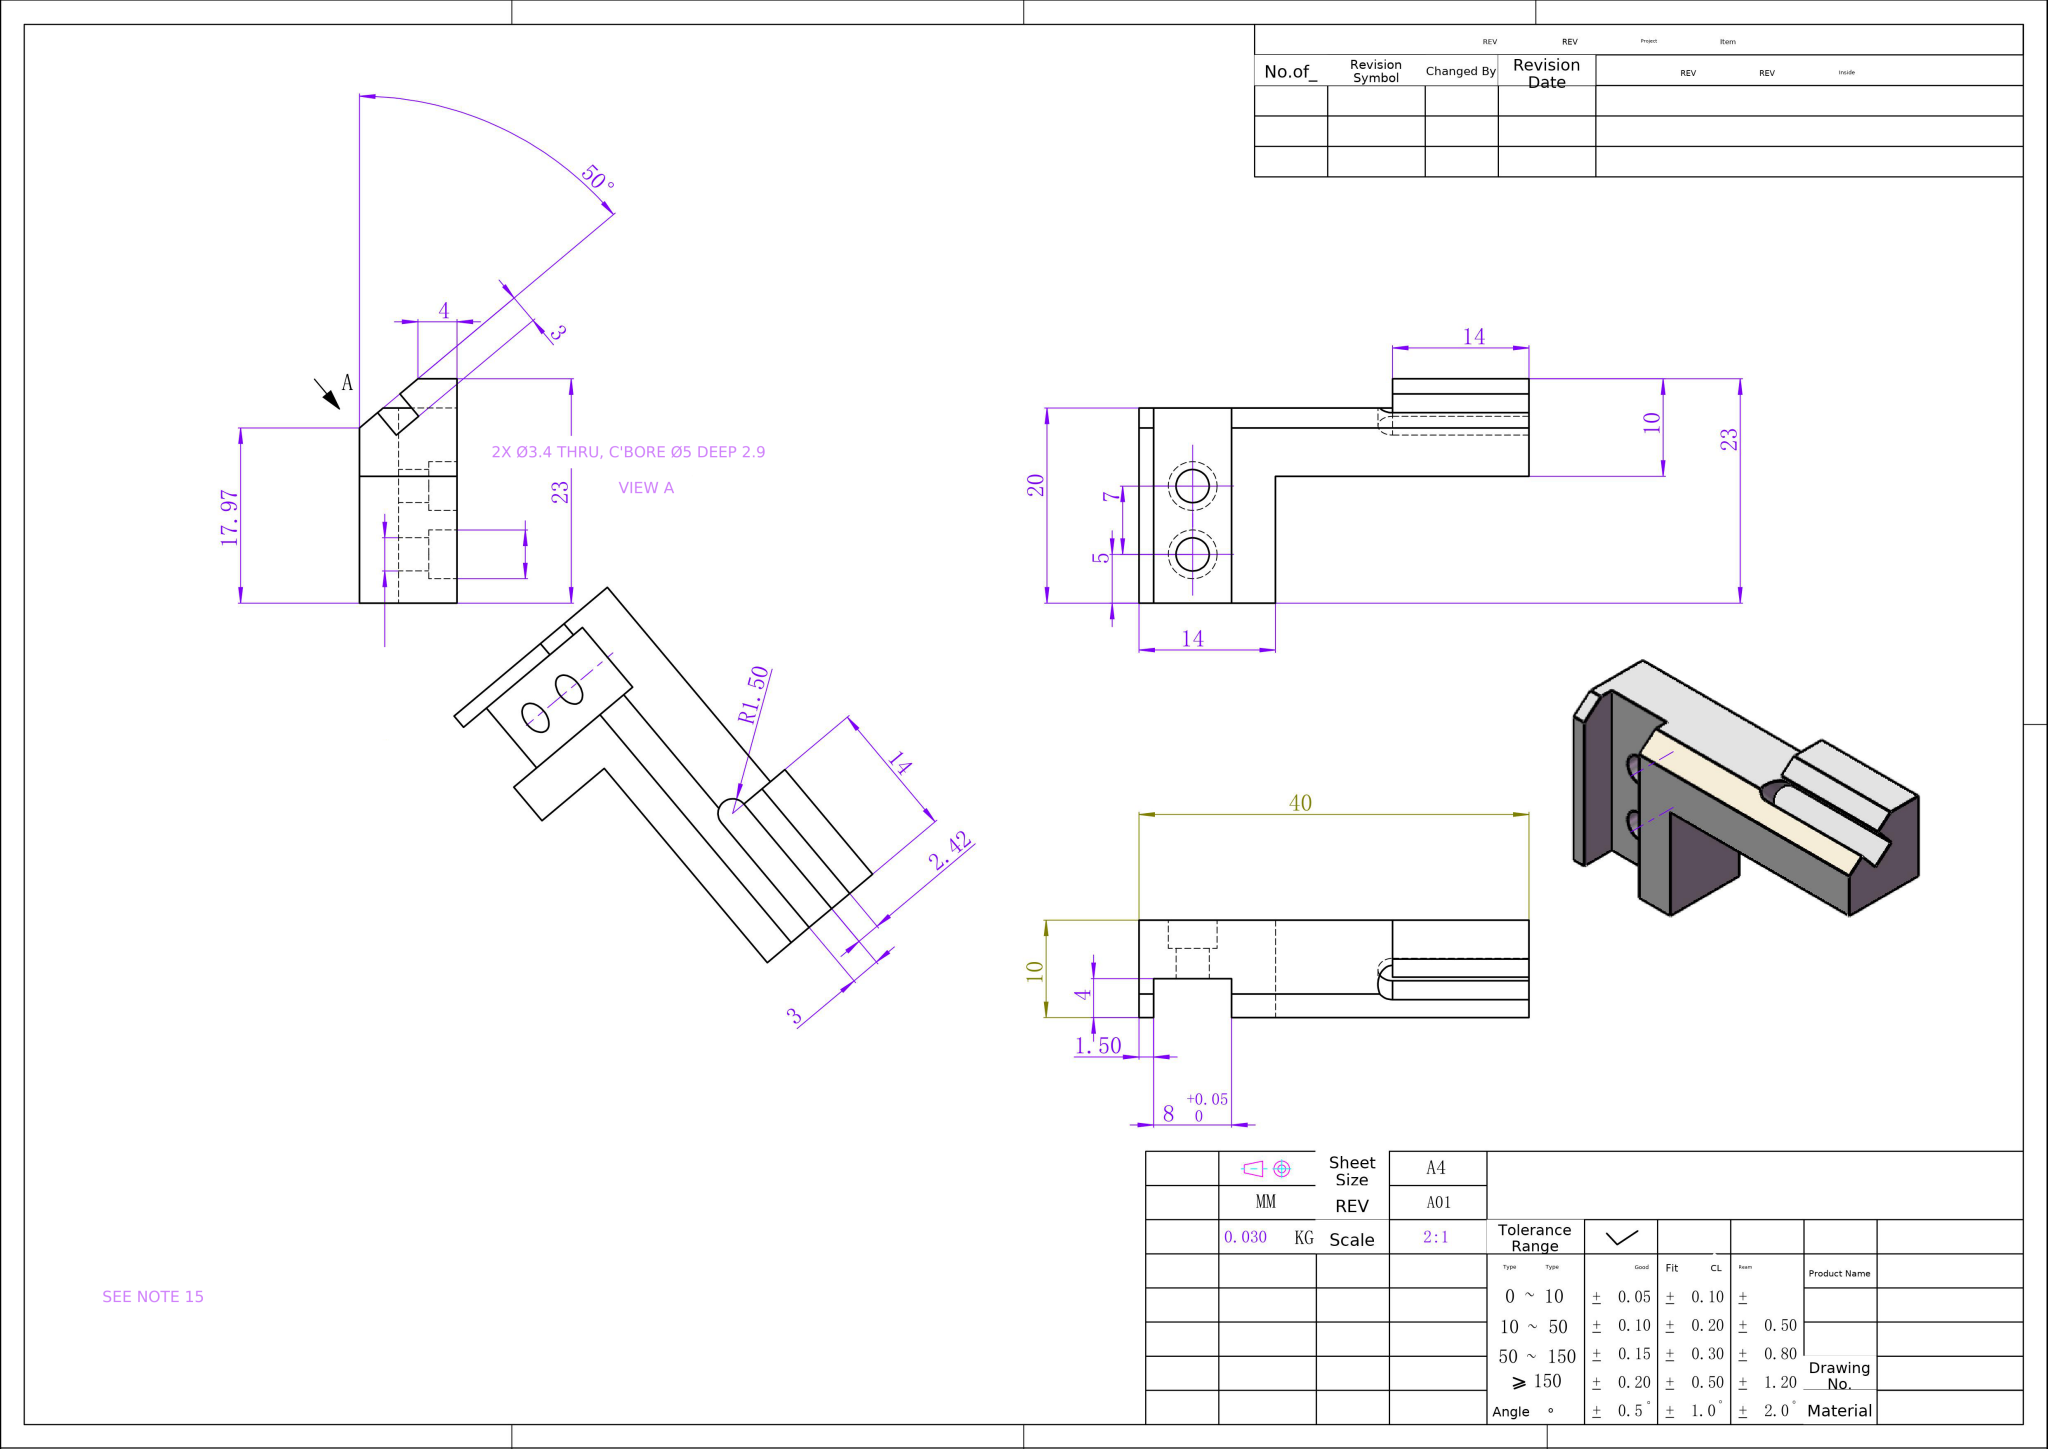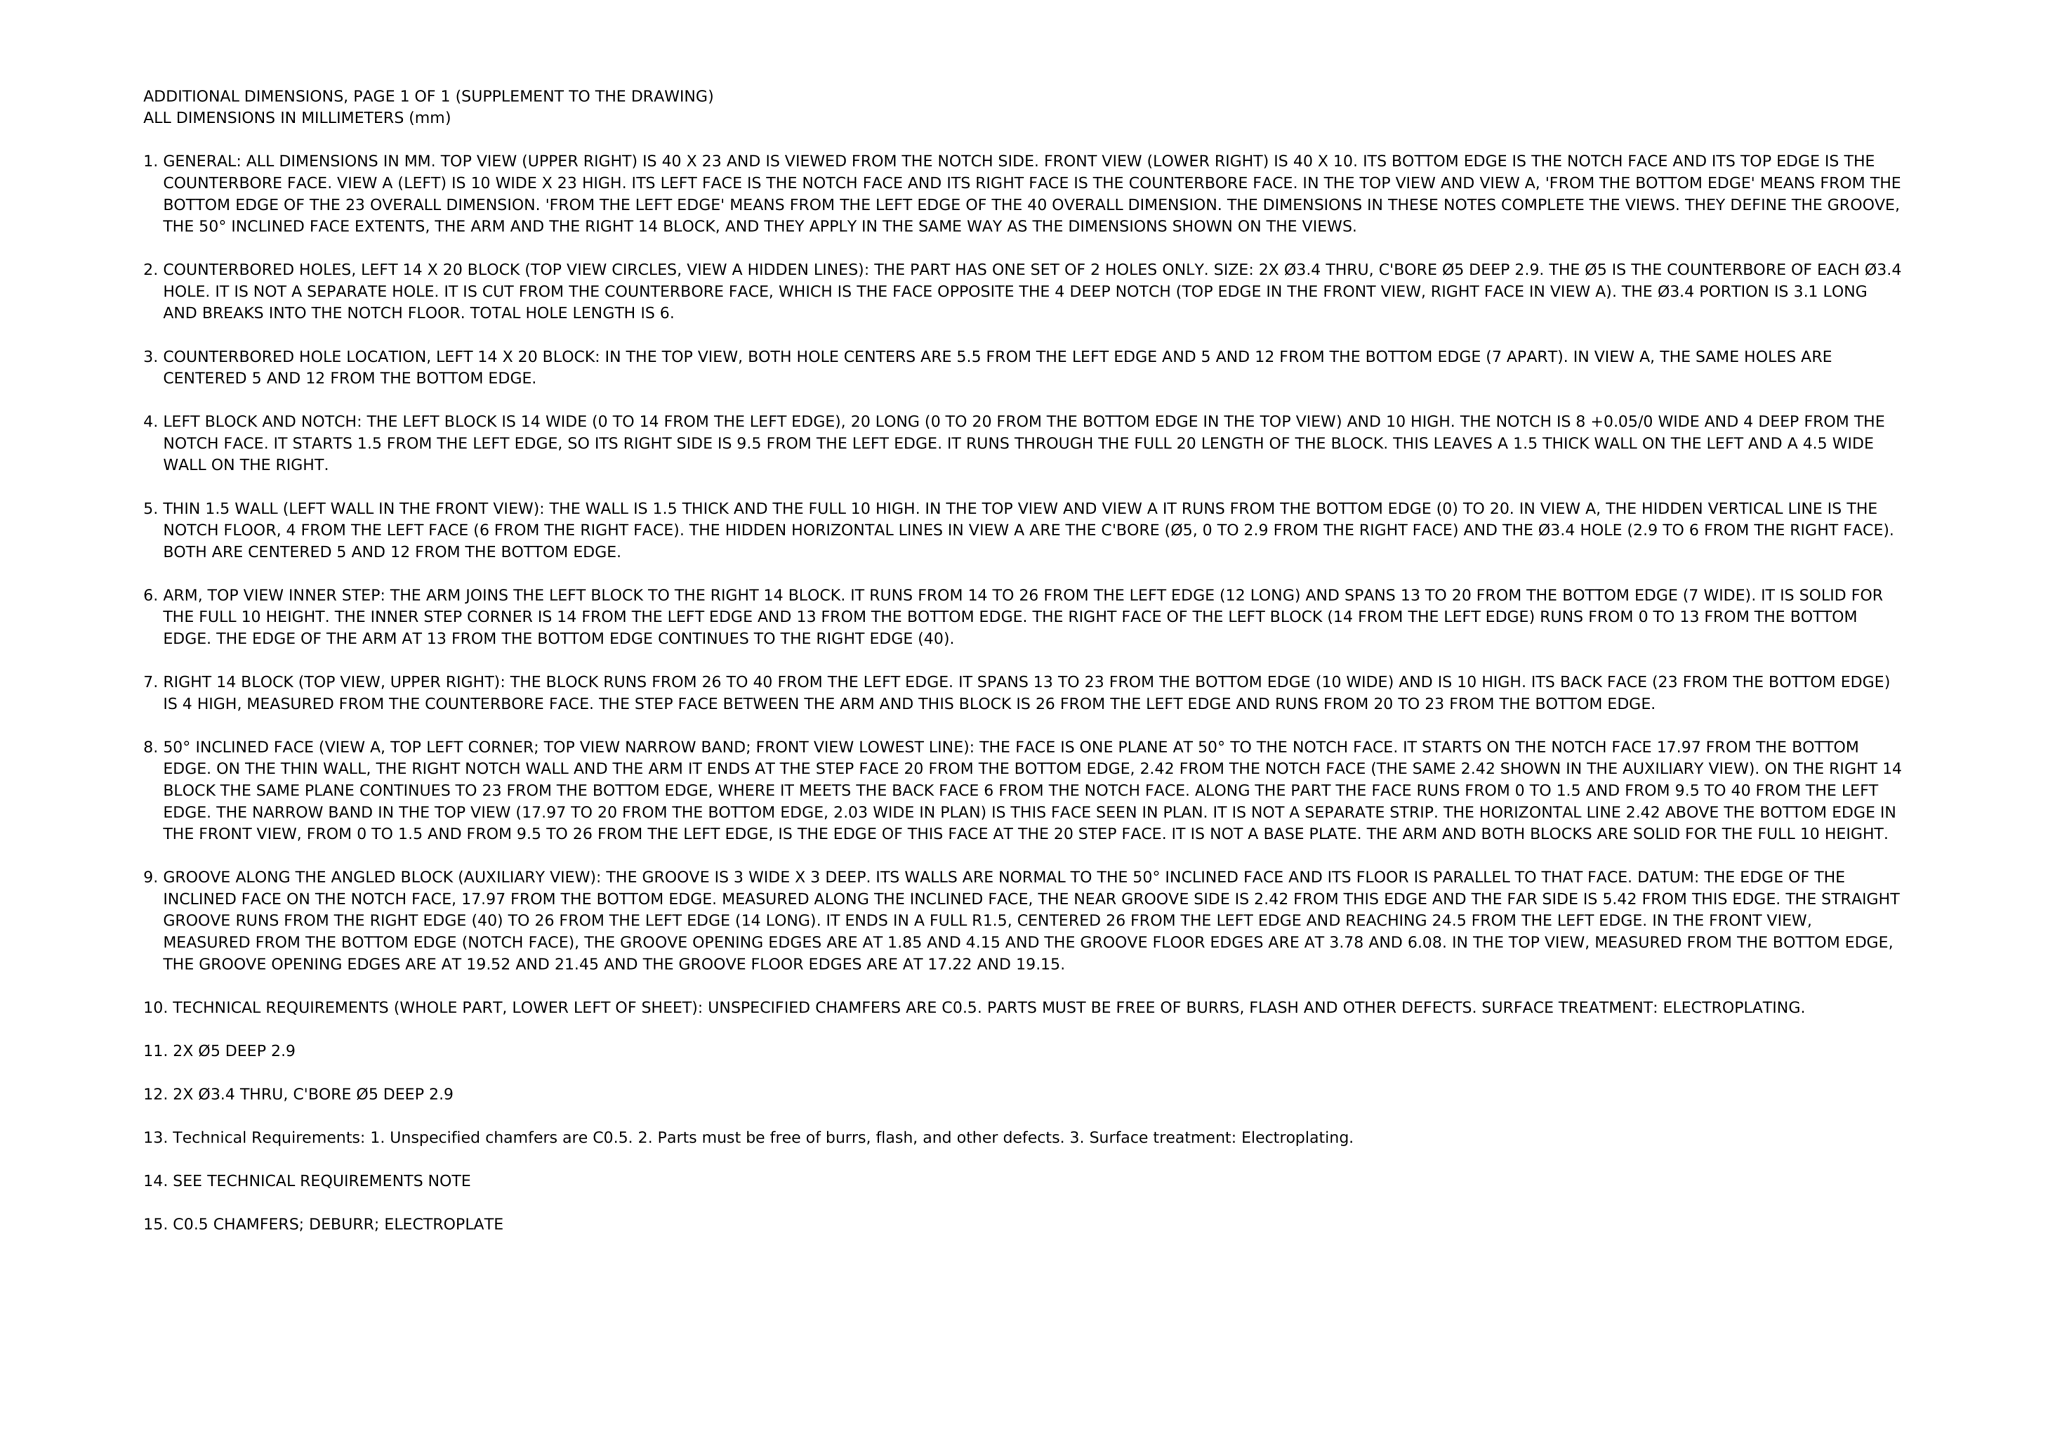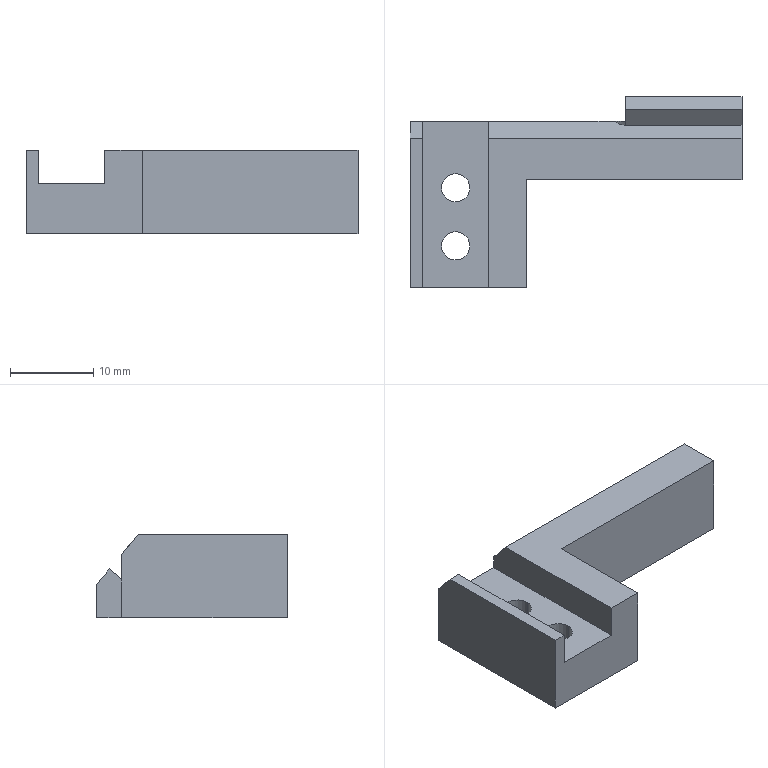Part | NX | mm | 1 solid | 31 faces | box 40 x 23 x 10 mm | volume 3840 mm3 | plane 22 | cylinder 9 | commonest cylinder face diameters 3.4 x4 5 x4 3 x1